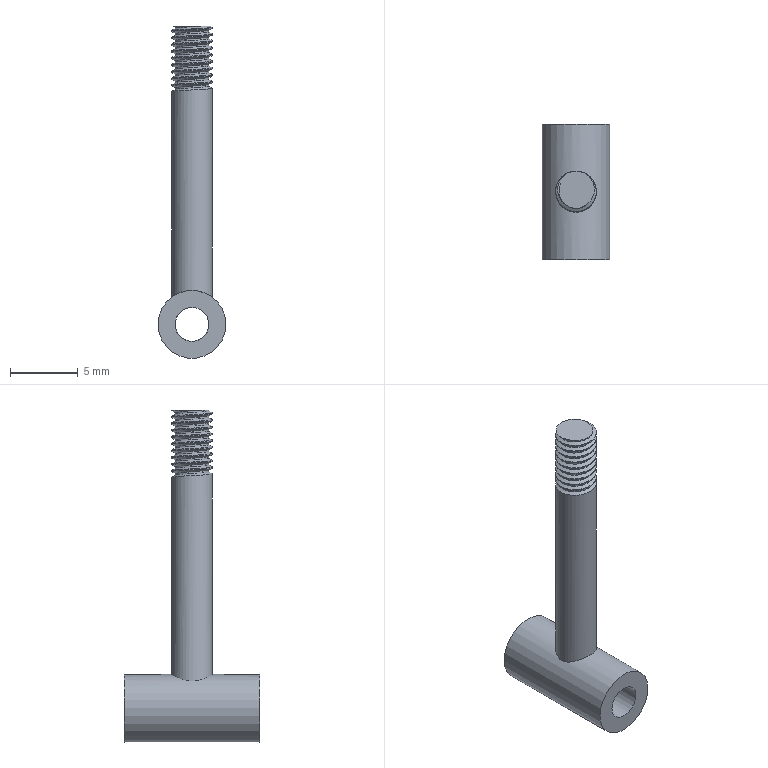Component | NX | LOCATING_POST | 1 solid | 19 faces | volume 280 mm3 | cylinder 13 | plane 4 | spline 2 | commonest cylinder face diameters 3 x10 2.5 x2 5 x1